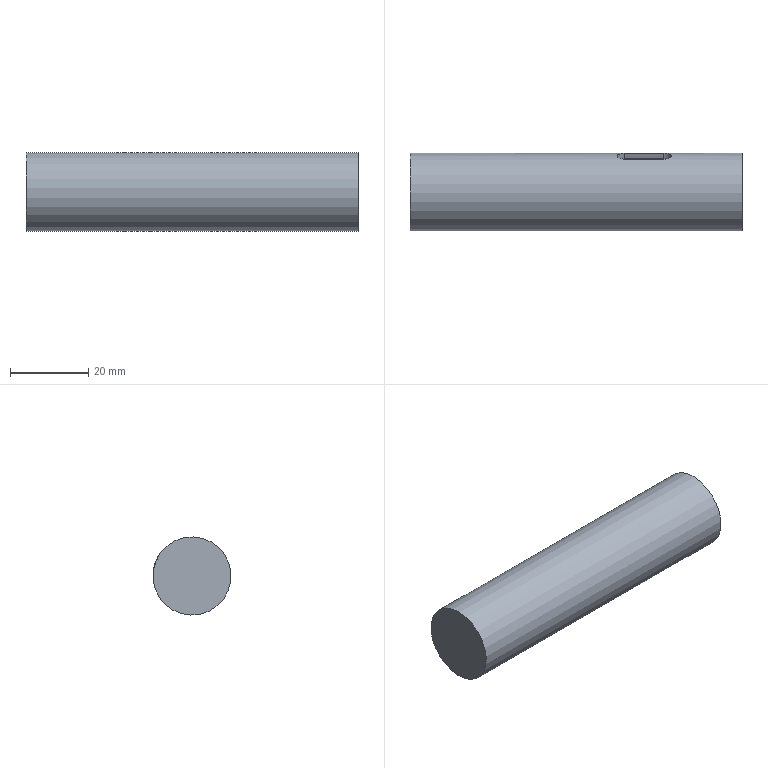Component | NX | CCJ-020 | 1 solid | 8 faces | box 85 x 20 x 20 mm | volume 26623 mm3 | plane 5 | cylinder 3 | commonest cylinder face diameters 4 x2 20 x1
STEP:
#1=CARTESIAN_POINT('',(0.,0.,0.));
#2=DIRECTION('',(0.,0.,1.));
#3=DIRECTION('',(1.,0.,0.));
#4=AXIS2_PLACEMENT_3D('',#1,#2,#3);
#5=CARTESIAN_POINT('',(26.329,34.242,-20.986));
#6=VERTEX_POINT('',#5);
#7=CARTESIAN_POINT('',(26.329,25.,-24.804));
#8=DIRECTION('',(-1.,0.,0.));
#9=DIRECTION('',(0.,0.9242,0.3818));
#10=AXIS2_PLACEMENT_3D('',#7,#8,#9);
#11=CIRCLE('',#10,10.);
#12=CARTESIAN_POINT('',(-58.671,25.,-24.804));
#13=DIRECTION('',(1.,0.,0.));
#14=DIRECTION('',(0.,-0.9242,-0.3818));
#15=AXIS2_PLACEMENT_3D('',#12,#13,#14);
#16=CYLINDRICAL_SURFACE('',#15,10.);
#17=CARTESIAN_POINT('',(9.425,85.));
#18=DIRECTION('',(-1.,0.));
#19=VECTOR('',#18,1.);
#20=LINE('',#17,#19);
#21=(GEOMETRIC_REPRESENTATION_CONTEXT(2)PARAMETRIC_REPRESENTATION_CONTEXT()REPRESENTATION_CONTEXT('',''));
#22=DEFINITIONAL_REPRESENTATION('',(#20),#21);
#23=PCURVE('',#16,#22);
#24=CARTESIAN_POINT('',(26.329,25.,-24.804));
#25=DIRECTION('',(-1.,0.,0.));
#26=DIRECTION('',(0.,0.9242,0.3818));
#27=AXIS2_PLACEMENT_3D('',#24,#25,#26);
#28=PLANE('',#27);
#29=CARTESIAN_POINT('',(0.,0.));
#30=DIRECTION('',(1.,0.));
#31=AXIS2_PLACEMENT_2D('',#29,#30);
#32=CIRCLE('',#31,10.);
#33=(GEOMETRIC_REPRESENTATION_CONTEXT(2)PARAMETRIC_REPRESENTATION_CONTEXT()REPRESENTATION_CONTEXT('',''));
#34=DEFINITIONAL_REPRESENTATION('',(#32),#33);
#35=PCURVE('',#28,#34);
#36=SURFACE_CURVE('',#11,(#23,#35),.PCURVE_S1.);
#37=EDGE_CURVE('',#6,#6,#36,.T.);
#38=ORIENTED_EDGE('',*,*,#37,.T.);
#39=CARTESIAN_POINT('',(8.329,34.242,-20.986));
#40=VERTEX_POINT('',#39);
#41=CARTESIAN_POINT('',(8.329,34.242,-20.986));
#42=CARTESIAN_POINT('',(26.329,34.242,-20.986));
#43=B_SPLINE_CURVE_WITH_KNOTS('',1,(#41,#42),.UNSPECIFIED.,.F.,.F.,(2,2),(67.,85.),.PIECEWISE_BEZIER_KNOTS.);
#44=CARTESIAN_POINT('',(3.142,0.));
#45=DIRECTION('',(0.,1.));
#46=VECTOR('',#45,1.);
#47=LINE('',#44,#46);
#48=(GEOMETRIC_REPRESENTATION_CONTEXT(2)PARAMETRIC_REPRESENTATION_CONTEXT()REPRESENTATION_CONTEXT('',''));
#49=DEFINITIONAL_REPRESENTATION('',(#47),#48);
#50=PCURVE('',#16,#49);
#51=CARTESIAN_POINT('',(9.425,0.));
#52=DIRECTION('',(0.,1.));
#53=VECTOR('',#52,1.);
#54=LINE('',#51,#53);
#55=(GEOMETRIC_REPRESENTATION_CONTEXT(2)PARAMETRIC_REPRESENTATION_CONTEXT()REPRESENTATION_CONTEXT('',''));
#56=DEFINITIONAL_REPRESENTATION('',(#54),#55);
#57=PCURVE('',#16,#56);
#58=SEAM_CURVE('',#43,(#50,#57),.PCURVE_S1.);
#59=EDGE_CURVE('',#40,#6,#58,.T.);
#60=ORIENTED_EDGE('',*,*,#59,.F.);
#61=CARTESIAN_POINT('',(6.329,33.292,-19.214));
#62=VERTEX_POINT('',#61);
#63=CARTESIAN_POINT('',(6.329,33.292,-19.214));
#64=CARTESIAN_POINT('',(6.55,33.292,-19.214));
#65=CARTESIAN_POINT('',(6.775,33.314,-19.246));
#66=CARTESIAN_POINT('',(6.983,33.354,-19.308));
#67=CARTESIAN_POINT('',(7.192,33.394,-19.369));
#68=CARTESIAN_POINT('',(7.391,33.455,-19.462));
#69=CARTESIAN_POINT('',(7.564,33.526,-19.579));
#70=CARTESIAN_POINT('',(7.739,33.599,-19.698));
#71=CARTESIAN_POINT('',(7.893,33.686,-19.846));
#72=CARTESIAN_POINT('',(8.014,33.777,-20.012));
#73=CARTESIAN_POINT('',(8.135,33.868,-20.179));
#74=CARTESIAN_POINT('',(8.225,33.966,-20.37));
#75=CARTESIAN_POINT('',(8.276,34.059,-20.569));
#76=CARTESIAN_POINT('',(8.327,34.151,-20.766));
#77=CARTESIAN_POINT('',(8.341,34.241,-20.976));
#78=CARTESIAN_POINT('',(8.318,34.321,-21.183));
#79=CARTESIAN_POINT('',(8.294,34.4,-21.387));
#80=CARTESIAN_POINT('',(8.234,34.472,-21.592));
#81=CARTESIAN_POINT('',(8.141,34.532,-21.782));
#82=CARTESIAN_POINT('',(8.047,34.593,-21.973));
#83=CARTESIAN_POINT('',(7.919,34.644,-22.154));
#84=CARTESIAN_POINT('',(7.766,34.684,-22.309));
#85=CARTESIAN_POINT('',(7.61,34.724,-22.466));
#86=CARTESIAN_POINT('',(7.424,34.755,-22.601));
#87=CARTESIAN_POINT('',(7.224,34.776,-22.7));
#88=CARTESIAN_POINT('',(7.023,34.798,-22.8));
#89=CARTESIAN_POINT('',(6.801,34.811,-22.868));
#90=CARTESIAN_POINT('',(6.577,34.816,-22.896));
#91=CARTESIAN_POINT('',(6.495,34.818,-22.906));
#92=CARTESIAN_POINT('',(6.412,34.819,-22.911));
#93=CARTESIAN_POINT('',(6.329,34.819,-22.911));
#94=B_SPLINE_CURVE_WITH_KNOTS('',3,(#63,#64,#65,#66,#67,#68,#69,#70,#71,#72,#73,#74,#75,#76,#77,#78,#79,#80,#81,#82,#83,#84,#85,#86,#87,#88,#89,#90,#91,#92,#93),.UNSPECIFIED.,.F.,.F.,(4,3,3,3,3,3,3,3,3,3,4),(0.,0.106,0.2118,0.319,0.4272,0.534,0.6392,0.745,0.8528,0.9608,1.),.UNSPECIFIED.);
#95=CARTESIAN_POINT('',(3.343,65.));
#96=CARTESIAN_POINT('',(3.343,65.047));
#97=CARTESIAN_POINT('',(3.343,65.143));
#98=CARTESIAN_POINT('',(3.341,65.285));
#99=CARTESIAN_POINT('',(3.338,65.427));
#100=CARTESIAN_POINT('',(3.335,65.565));
#101=CARTESIAN_POINT('',(3.33,65.7));
#102=CARTESIAN_POINT('',(3.325,65.832));
#103=CARTESIAN_POINT('',(3.318,65.96));
#104=CARTESIAN_POINT('',(3.311,66.083));
#105=CARTESIAN_POINT('',(3.302,66.2));
#106=CARTESIAN_POINT('',(3.293,66.31));
#107=CARTESIAN_POINT('',(3.284,66.415));
#108=CARTESIAN_POINT('',(3.273,66.512));
#109=CARTESIAN_POINT('',(3.262,66.602));
#110=CARTESIAN_POINT('',(3.25,66.683));
#111=CARTESIAN_POINT('',(3.238,66.756));
#112=CARTESIAN_POINT('',(3.225,66.82));
#113=CARTESIAN_POINT('',(3.212,66.875));
#114=CARTESIAN_POINT('',(3.198,66.92));
#115=CARTESIAN_POINT('',(3.184,66.956));
#116=CARTESIAN_POINT('',(3.17,66.981));
#117=CARTESIAN_POINT('',(3.156,66.996));
#118=CARTESIAN_POINT('',(3.142,67.002));
#119=CARTESIAN_POINT('',(3.127,66.997));
#120=CARTESIAN_POINT('',(3.113,66.981));
#121=CARTESIAN_POINT('',(3.099,66.956));
#122=CARTESIAN_POINT('',(3.085,66.92));
#123=CARTESIAN_POINT('',(3.072,66.875));
#124=CARTESIAN_POINT('',(3.058,66.821));
#125=CARTESIAN_POINT('',(3.046,66.757));
#126=CARTESIAN_POINT('',(3.033,66.684));
#127=CARTESIAN_POINT('',(3.021,66.603));
#128=CARTESIAN_POINT('',(3.01,66.513));
#129=CARTESIAN_POINT('',(3.,66.416));
#130=CARTESIAN_POINT('',(2.99,66.312));
#131=CARTESIAN_POINT('',(2.981,66.201));
#132=CARTESIAN_POINT('',(2.973,66.084));
#133=CARTESIAN_POINT('',(2.965,65.961));
#134=CARTESIAN_POINT('',(2.959,65.834));
#135=CARTESIAN_POINT('',(2.953,65.703));
#136=CARTESIAN_POINT('',(2.948,65.567));
#137=CARTESIAN_POINT('',(2.945,65.428));
#138=CARTESIAN_POINT('',(2.942,65.288));
#139=CARTESIAN_POINT('',(2.941,65.144));
#140=CARTESIAN_POINT('',(2.94,65.048));
#141=CARTESIAN_POINT('',(2.94,65.));
#142=B_SPLINE_CURVE_WITH_KNOTS('',3,(#95,#96,#97,#98,#99,#100,#101,#102,#103,#104,#105,#106,#107,#108,#109,#110,#111,#112,#113,#114,#115,#116,#117,#118,#119,#120,#121,#122,#123,#124,#125,#126,#127,#128,#129,#130,#131,#132,#133,#134,#135,#136,#137,#138,#139,#140,#141),.UNSPECIFIED.,.F.,.F.,(4,1,1,1,1,1,1,1,1,1,1,1,1,1,1,1,1,1,1,1,1,1,1,1,1,1,1,1,1,1,1,1,1,1,1,1,1,1,1,1,1,1,1,1,4),(0.,0.02273,0.04545,0.06818,0.09091,0.1136,0.1364,0.1591,0.1818,0.2045,0.2273,0.25,0.2727,0.2955,0.3182,0.3409,0.3636,0.3864,0.4091,0.4318,0.4545,0.4773,0.5,0.5227,0.5455,0.5682,0.5909,0.6136,0.6364,0.6591,0.6818,0.7045,0.7273,0.75,0.7727,0.7955,0.8182,0.8409,0.8636,0.8864,0.9091,0.9318,0.9545,0.9773,1.),.QUASI_UNIFORM_KNOTS.);
#143=(GEOMETRIC_REPRESENTATION_CONTEXT(2)PARAMETRIC_REPRESENTATION_CONTEXT()REPRESENTATION_CONTEXT('',''));
#144=DEFINITIONAL_REPRESENTATION('',(#142),#143);
#145=PCURVE('',#16,#144);
#146=CARTESIAN_POINT('',(6.329,38.863,-19.077));
#147=DIRECTION('',(0.,-0.9242,-0.3818));
#148=DIRECTION('',(-1.,0.,0.));
#149=AXIS2_PLACEMENT_3D('',#146,#147,#148);
#150=CYLINDRICAL_SURFACE('',#149,2.);
#151=CARTESIAN_POINT('',(4.712,5.202));
#152=CARTESIAN_POINT('',(3.142,5.));
#153=B_SPLINE_CURVE_WITH_KNOTS('',1,(#151,#152),.UNSPECIFIED.,.F.,.F.,(2,2),(0.,0.5001),.PIECEWISE_BEZIER_KNOTS.);
#154=(GEOMETRIC_REPRESENTATION_CONTEXT(2)PARAMETRIC_REPRESENTATION_CONTEXT()REPRESENTATION_CONTEXT('',''));
#155=DEFINITIONAL_REPRESENTATION('',(#153),#154);
#156=PCURVE('',#150,#155);
#157=SURFACE_CURVE('',#94,(#145,#156),.PCURVE_S1.);
#158=EDGE_CURVE('',#62,#40,#157,.T.);
#159=ORIENTED_EDGE('',*,*,#158,.F.);
#160=CARTESIAN_POINT('',(-3.671,33.292,-19.214));
#161=VERTEX_POINT('',#160);
#162=CARTESIAN_POINT('',(-58.671,33.292,-19.214));
#163=DIRECTION('',(1.,0.,0.));
#164=VECTOR('',#163,1.);
#165=LINE('',#162,#164);
#166=CARTESIAN_POINT('',(3.343,0.));
#167=DIRECTION('',(0.,1.));
#168=VECTOR('',#167,1.);
#169=LINE('',#166,#168);
#170=(GEOMETRIC_REPRESENTATION_CONTEXT(2)PARAMETRIC_REPRESENTATION_CONTEXT()REPRESENTATION_CONTEXT('',''));
#171=DEFINITIONAL_REPRESENTATION('',(#169),#170);
#172=PCURVE('',#16,#171);
#173=CARTESIAN_POINT('',(-3.671,38.1,-17.228));
#174=DIRECTION('',(0.,0.3818,-0.9242));
#175=DIRECTION('',(-1.,0.,0.));
#176=AXIS2_PLACEMENT_3D('',#173,#174,#175);
#177=PLANE('',#176);
#178=CARTESIAN_POINT('',(55.,-5.202));
#179=DIRECTION('',(-1.,0.));
#180=VECTOR('',#179,1.);
#181=LINE('',#178,#180);
#182=(GEOMETRIC_REPRESENTATION_CONTEXT(2)PARAMETRIC_REPRESENTATION_CONTEXT()REPRESENTATION_CONTEXT('',''));
#183=DEFINITIONAL_REPRESENTATION('',(#181),#182);
#184=PCURVE('',#177,#183);
#185=SURFACE_CURVE('',#165,(#172,#184),.PCURVE_S1.);
#186=EDGE_CURVE('',#161,#62,#185,.T.);
#187=ORIENTED_EDGE('',*,*,#186,.F.);
#188=CARTESIAN_POINT('',(-5.671,34.242,-20.986));
#189=VERTEX_POINT('',#188);
#190=CARTESIAN_POINT('',(-3.671,34.819,-22.911));
#191=CARTESIAN_POINT('',(-3.892,34.819,-22.911));
#192=CARTESIAN_POINT('',(-4.117,34.812,-22.873));
#193=CARTESIAN_POINT('',(-4.326,34.797,-22.801));
#194=CARTESIAN_POINT('',(-4.534,34.783,-22.729));
#195=CARTESIAN_POINT('',(-4.733,34.76,-22.621));
#196=CARTESIAN_POINT('',(-4.906,34.728,-22.487));
#197=CARTESIAN_POINT('',(-5.082,34.696,-22.352));
#198=CARTESIAN_POINT('',(-5.236,34.653,-22.186));
#199=CARTESIAN_POINT('',(-5.356,34.6,-22.004));
#200=CARTESIAN_POINT('',(-5.477,34.547,-21.821));
#201=CARTESIAN_POINT('',(-5.567,34.481,-21.617));
#202=CARTESIAN_POINT('',(-5.619,34.406,-21.41));
#203=CARTESIAN_POINT('',(-5.669,34.333,-21.206));
#204=CARTESIAN_POINT('',(-5.683,34.248,-20.993));
#205=CARTESIAN_POINT('',(-5.66,34.159,-20.79));
#206=CARTESIAN_POINT('',(-5.636,34.071,-20.59));
#207=CARTESIAN_POINT('',(-5.576,33.977,-20.394));
#208=CARTESIAN_POINT('',(-5.483,33.886,-20.217));
#209=CARTESIAN_POINT('',(-5.39,33.794,-20.039));
#210=CARTESIAN_POINT('',(-5.261,33.702,-19.875));
#211=CARTESIAN_POINT('',(-5.108,33.621,-19.737));
#212=CARTESIAN_POINT('',(-4.952,33.539,-19.597));
#213=CARTESIAN_POINT('',(-4.767,33.465,-19.48));
#214=CARTESIAN_POINT('',(-4.566,33.41,-19.394));
#215=CARTESIAN_POINT('',(-4.365,33.355,-19.308));
#216=CARTESIAN_POINT('',(-4.143,33.317,-19.251));
#217=CARTESIAN_POINT('',(-3.92,33.301,-19.228));
#218=CARTESIAN_POINT('',(-3.837,33.295,-19.219));
#219=CARTESIAN_POINT('',(-3.754,33.292,-19.214));
#220=CARTESIAN_POINT('',(-3.671,33.292,-19.214));
#221=B_SPLINE_CURVE_WITH_KNOTS('',3,(#190,#191,#192,#193,#194,#195,#196,#197,#198,#199,#200,#201,#202,#203,#204,#205,#206,#207,#208,#209,#210,#211,#212,#213,#214,#215,#216,#217,#218,#219,#220),.UNSPECIFIED.,.F.,.F.,(4,3,3,3,3,3,3,3,3,3,4),(0.,0.106,0.2118,0.319,0.4272,0.534,0.6392,0.745,0.8528,0.9608,1.),.UNSPECIFIED.);
#222=CARTESIAN_POINT('',(2.94,55.));
#223=CARTESIAN_POINT('',(2.94,54.953));
#224=CARTESIAN_POINT('',(2.941,54.857));
#225=CARTESIAN_POINT('',(2.942,54.715));
#226=CARTESIAN_POINT('',(2.945,54.573));
#227=CARTESIAN_POINT('',(2.948,54.435));
#228=CARTESIAN_POINT('',(2.953,54.3));
#229=CARTESIAN_POINT('',(2.959,54.168));
#230=CARTESIAN_POINT('',(2.965,54.04));
#231=CARTESIAN_POINT('',(2.972,53.917));
#232=CARTESIAN_POINT('',(2.981,53.8));
#233=CARTESIAN_POINT('',(2.99,53.69));
#234=CARTESIAN_POINT('',(3.,53.585));
#235=CARTESIAN_POINT('',(3.01,53.488));
#236=CARTESIAN_POINT('',(3.021,53.398));
#237=CARTESIAN_POINT('',(3.033,53.317));
#238=CARTESIAN_POINT('',(3.045,53.244));
#239=CARTESIAN_POINT('',(3.058,53.18));
#240=CARTESIAN_POINT('',(3.071,53.125));
#241=CARTESIAN_POINT('',(3.085,53.08));
#242=CARTESIAN_POINT('',(3.099,53.044));
#243=CARTESIAN_POINT('',(3.113,53.019));
#244=CARTESIAN_POINT('',(3.127,53.004));
#245=CARTESIAN_POINT('',(3.142,52.998));
#246=CARTESIAN_POINT('',(3.156,53.003));
#247=CARTESIAN_POINT('',(3.17,53.019));
#248=CARTESIAN_POINT('',(3.184,53.044));
#249=CARTESIAN_POINT('',(3.198,53.08));
#250=CARTESIAN_POINT('',(3.212,53.125));
#251=CARTESIAN_POINT('',(3.225,53.179));
#252=CARTESIAN_POINT('',(3.238,53.243));
#253=CARTESIAN_POINT('',(3.25,53.316));
#254=CARTESIAN_POINT('',(3.262,53.397));
#255=CARTESIAN_POINT('',(3.273,53.487));
#256=CARTESIAN_POINT('',(3.284,53.584));
#257=CARTESIAN_POINT('',(3.293,53.688));
#258=CARTESIAN_POINT('',(3.302,53.799));
#259=CARTESIAN_POINT('',(3.311,53.916));
#260=CARTESIAN_POINT('',(3.318,54.039));
#261=CARTESIAN_POINT('',(3.325,54.166));
#262=CARTESIAN_POINT('',(3.33,54.297));
#263=CARTESIAN_POINT('',(3.335,54.433));
#264=CARTESIAN_POINT('',(3.338,54.572));
#265=CARTESIAN_POINT('',(3.341,54.712));
#266=CARTESIAN_POINT('',(3.343,54.856));
#267=CARTESIAN_POINT('',(3.343,54.952));
#268=CARTESIAN_POINT('',(3.343,55.));
#269=B_SPLINE_CURVE_WITH_KNOTS('',3,(#222,#223,#224,#225,#226,#227,#228,#229,#230,#231,#232,#233,#234,#235,#236,#237,#238,#239,#240,#241,#242,#243,#244,#245,#246,#247,#248,#249,#250,#251,#252,#253,#254,#255,#256,#257,#258,#259,#260,#261,#262,#263,#264,#265,#266,#267,#268),.UNSPECIFIED.,.F.,.F.,(4,1,1,1,1,1,1,1,1,1,1,1,1,1,1,1,1,1,1,1,1,1,1,1,1,1,1,1,1,1,1,1,1,1,1,1,1,1,1,1,1,1,1,1,4),(0.,0.02273,0.04545,0.06818,0.09091,0.1136,0.1364,0.1591,0.1818,0.2045,0.2273,0.25,0.2727,0.2955,0.3182,0.3409,0.3636,0.3864,0.4091,0.4318,0.4545,0.4773,0.5,0.5227,0.5455,0.5682,0.5909,0.6136,0.6364,0.6591,0.6818,0.7045,0.7273,0.75,0.7727,0.7955,0.8182,0.8409,0.8636,0.8864,0.9091,0.9318,0.9545,0.9773,1.),.QUASI_UNIFORM_KNOTS.);
#270=(GEOMETRIC_REPRESENTATION_CONTEXT(2)PARAMETRIC_REPRESENTATION_CONTEXT()REPRESENTATION_CONTEXT('',''));
#271=DEFINITIONAL_REPRESENTATION('',(#269),#270);
#272=PCURVE('',#16,#271);
#273=CARTESIAN_POINT('',(-3.671,38.863,-19.077));
#274=DIRECTION('',(0.,-0.9242,-0.3818));
#275=DIRECTION('',(-1.,0.,0.));
#276=AXIS2_PLACEMENT_3D('',#273,#274,#275);
#277=CYLINDRICAL_SURFACE('',#276,2.);
#278=CARTESIAN_POINT('',(0.00000002,5.));
#279=CARTESIAN_POINT('',(-1.571,5.202));
#280=B_SPLINE_CURVE_WITH_KNOTS('',1,(#278,#279),.UNSPECIFIED.,.F.,.F.,(2,2),(0.5001,1.),.PIECEWISE_BEZIER_KNOTS.);
#281=(GEOMETRIC_REPRESENTATION_CONTEXT(2)PARAMETRIC_REPRESENTATION_CONTEXT()REPRESENTATION_CONTEXT('',''));
#282=DEFINITIONAL_REPRESENTATION('',(#280),#281);
#283=PCURVE('',#277,#282);
#284=SURFACE_CURVE('',#221,(#272,#283),.PCURVE_S1.);
#285=EDGE_CURVE('',#189,#161,#284,.T.);
#286=ORIENTED_EDGE('',*,*,#285,.F.);
#287=CARTESIAN_POINT('',(-58.671,34.242,-20.986));
#288=VERTEX_POINT('',#287);
#289=CARTESIAN_POINT('',(-58.671,34.242,-20.986));
#290=CARTESIAN_POINT('',(-5.671,34.242,-20.986));
#291=B_SPLINE_CURVE_WITH_KNOTS('',1,(#289,#290),.UNSPECIFIED.,.F.,.F.,(2,2),(0.,53.),.PIECEWISE_BEZIER_KNOTS.);
#292=CARTESIAN_POINT('',(3.142,0.));
#293=DIRECTION('',(0.,1.));
#294=VECTOR('',#293,1.);
#295=LINE('',#292,#294);
#296=(GEOMETRIC_REPRESENTATION_CONTEXT(2)PARAMETRIC_REPRESENTATION_CONTEXT()REPRESENTATION_CONTEXT('',''));
#297=DEFINITIONAL_REPRESENTATION('',(#295),#296);
#298=PCURVE('',#16,#297);
#299=CARTESIAN_POINT('',(9.425,0.));
#300=DIRECTION('',(0.,1.));
#301=VECTOR('',#300,1.);
#302=LINE('',#299,#301);
#303=(GEOMETRIC_REPRESENTATION_CONTEXT(2)PARAMETRIC_REPRESENTATION_CONTEXT()REPRESENTATION_CONTEXT('',''));
#304=DEFINITIONAL_REPRESENTATION('',(#302),#303);
#305=PCURVE('',#16,#304);
#306=SEAM_CURVE('',#291,(#298,#305),.PCURVE_S1.);
#307=EDGE_CURVE('',#288,#189,#306,.T.);
#308=ORIENTED_EDGE('',*,*,#307,.F.);
#309=CARTESIAN_POINT('',(-58.671,25.,-24.804));
#310=DIRECTION('',(-1.,0.,0.));
#311=DIRECTION('',(0.,0.9242,0.3818));
#312=AXIS2_PLACEMENT_3D('',#309,#310,#311);
#313=CIRCLE('',#312,10.);
#314=CARTESIAN_POINT('',(9.425,0.));
#315=DIRECTION('',(-1.,0.));
#316=VECTOR('',#315,1.);
#317=LINE('',#314,#316);
#318=(GEOMETRIC_REPRESENTATION_CONTEXT(2)PARAMETRIC_REPRESENTATION_CONTEXT()REPRESENTATION_CONTEXT('',''));
#319=DEFINITIONAL_REPRESENTATION('',(#317),#318);
#320=PCURVE('',#16,#319);
#321=CARTESIAN_POINT('',(-58.671,25.,-24.804));
#322=DIRECTION('',(-1.,0.,0.));
#323=DIRECTION('',(0.,0.9242,0.3818));
#324=AXIS2_PLACEMENT_3D('',#321,#322,#323);
#325=PLANE('',#324);
#326=CARTESIAN_POINT('',(0.,0.));
#327=DIRECTION('',(1.,0.));
#328=AXIS2_PLACEMENT_2D('',#326,#327);
#329=CIRCLE('',#328,10.);
#330=(GEOMETRIC_REPRESENTATION_CONTEXT(2)PARAMETRIC_REPRESENTATION_CONTEXT()REPRESENTATION_CONTEXT('',''));
#331=DEFINITIONAL_REPRESENTATION('',(#329),#330);
#332=PCURVE('',#325,#331);
#333=SURFACE_CURVE('',#313,(#320,#332),.PCURVE_S1.);
#334=EDGE_CURVE('',#288,#288,#333,.T.);
#335=ORIENTED_EDGE('',*,*,#334,.F.);
#336=ORIENTED_EDGE('',*,*,#307,.T.);
#337=CARTESIAN_POINT('',(-3.671,34.819,-22.911));
#338=VERTEX_POINT('',#337);
#339=CARTESIAN_POINT('',(-3.671,34.819,-22.911));
#340=CARTESIAN_POINT('',(-3.892,34.819,-22.911));
#341=CARTESIAN_POINT('',(-4.117,34.812,-22.873));
#342=CARTESIAN_POINT('',(-4.326,34.797,-22.801));
#343=CARTESIAN_POINT('',(-4.534,34.783,-22.729));
#344=CARTESIAN_POINT('',(-4.733,34.76,-22.621));
#345=CARTESIAN_POINT('',(-4.906,34.728,-22.487));
#346=CARTESIAN_POINT('',(-5.082,34.696,-22.352));
#347=CARTESIAN_POINT('',(-5.236,34.653,-22.186));
#348=CARTESIAN_POINT('',(-5.356,34.6,-22.004));
#349=CARTESIAN_POINT('',(-5.477,34.547,-21.821));
#350=CARTESIAN_POINT('',(-5.567,34.481,-21.617));
#351=CARTESIAN_POINT('',(-5.619,34.406,-21.41));
#352=CARTESIAN_POINT('',(-5.669,34.333,-21.206));
#353=CARTESIAN_POINT('',(-5.683,34.248,-20.993));
#354=CARTESIAN_POINT('',(-5.66,34.159,-20.79));
#355=CARTESIAN_POINT('',(-5.636,34.071,-20.59));
#356=CARTESIAN_POINT('',(-5.576,33.977,-20.394));
#357=CARTESIAN_POINT('',(-5.483,33.886,-20.217));
#358=CARTESIAN_POINT('',(-5.39,33.794,-20.039));
#359=CARTESIAN_POINT('',(-5.261,33.702,-19.875));
#360=CARTESIAN_POINT('',(-5.108,33.621,-19.737));
#361=CARTESIAN_POINT('',(-4.952,33.539,-19.597));
#362=CARTESIAN_POINT('',(-4.767,33.465,-19.48));
#363=CARTESIAN_POINT('',(-4.566,33.41,-19.394));
#364=CARTESIAN_POINT('',(-4.365,33.355,-19.308));
#365=CARTESIAN_POINT('',(-4.143,33.317,-19.251));
#366=CARTESIAN_POINT('',(-3.92,33.301,-19.228));
#367=CARTESIAN_POINT('',(-3.837,33.295,-19.219));
#368=CARTESIAN_POINT('',(-3.754,33.292,-19.214));
#369=CARTESIAN_POINT('',(-3.671,33.292,-19.214));
#370=B_SPLINE_CURVE_WITH_KNOTS('',3,(#339,#340,#341,#342,#343,#344,#345,#346,#347,#348,#349,#350,#351,#352,#353,#354,#355,#356,#357,#358,#359,#360,#361,#362,#363,#364,#365,#366,#367,#368,#369),.UNSPECIFIED.,.F.,.F.,(4,3,3,3,3,3,3,3,3,3,4),(0.,0.106,0.2118,0.319,0.4272,0.534,0.6392,0.745,0.8528,0.9608,1.),.UNSPECIFIED.);
#371=CARTESIAN_POINT('',(9.223,55.));
#372=CARTESIAN_POINT('',(9.223,54.953));
#373=CARTESIAN_POINT('',(9.224,54.857));
#374=CARTESIAN_POINT('',(9.225,54.715));
#375=CARTESIAN_POINT('',(9.228,54.573));
#376=CARTESIAN_POINT('',(9.232,54.435));
#377=CARTESIAN_POINT('',(9.236,54.3));
#378=CARTESIAN_POINT('',(9.242,54.168));
#379=CARTESIAN_POINT('',(9.248,54.04));
#380=CARTESIAN_POINT('',(9.256,53.917));
#381=CARTESIAN_POINT('',(9.264,53.8));
#382=CARTESIAN_POINT('',(9.273,53.69));
#383=CARTESIAN_POINT('',(9.283,53.585));
#384=CARTESIAN_POINT('',(9.293,53.488));
#385=CARTESIAN_POINT('',(9.304,53.398));
#386=CARTESIAN_POINT('',(9.316,53.317));
#387=CARTESIAN_POINT('',(9.329,53.244));
#388=CARTESIAN_POINT('',(9.341,53.18));
#389=CARTESIAN_POINT('',(9.355,53.125));
#390=CARTESIAN_POINT('',(9.368,53.08));
#391=CARTESIAN_POINT('',(9.382,53.044));
#392=CARTESIAN_POINT('',(9.396,53.019));
#393=CARTESIAN_POINT('',(9.41,53.004));
#394=CARTESIAN_POINT('',(9.425,52.998));
#395=CARTESIAN_POINT('',(9.439,53.003));
#396=CARTESIAN_POINT('',(9.453,53.019));
#397=CARTESIAN_POINT('',(9.467,53.044));
#398=CARTESIAN_POINT('',(9.481,53.08));
#399=CARTESIAN_POINT('',(9.495,53.125));
#400=CARTESIAN_POINT('',(9.508,53.179));
#401=CARTESIAN_POINT('',(9.521,53.243));
#402=CARTESIAN_POINT('',(9.533,53.316));
#403=CARTESIAN_POINT('',(9.545,53.397));
#404=CARTESIAN_POINT('',(9.556,53.487));
#405=CARTESIAN_POINT('',(9.567,53.584));
#406=CARTESIAN_POINT('',(9.576,53.688));
#407=CARTESIAN_POINT('',(9.586,53.799));
#408=CARTESIAN_POINT('',(9.594,53.916));
#409=CARTESIAN_POINT('',(9.601,54.039));
#410=CARTESIAN_POINT('',(9.608,54.166));
#411=CARTESIAN_POINT('',(9.613,54.297));
#412=CARTESIAN_POINT('',(9.618,54.433));
#413=CARTESIAN_POINT('',(9.622,54.572));
#414=CARTESIAN_POINT('',(9.624,54.712));
#415=CARTESIAN_POINT('',(9.626,54.856));
#416=CARTESIAN_POINT('',(9.626,54.952));
#417=CARTESIAN_POINT('',(9.626,55.));
#418=B_SPLINE_CURVE_WITH_KNOTS('',3,(#371,#372,#373,#374,#375,#376,#377,#378,#379,#380,#381,#382,#383,#384,#385,#386,#387,#388,#389,#390,#391,#392,#393,#394,#395,#396,#397,#398,#399,#400,#401,#402,#403,#404,#405,#406,#407,#408,#409,#410,#411,#412,#413,#414,#415,#416,#417),.UNSPECIFIED.,.F.,.F.,(4,1,1,1,1,1,1,1,1,1,1,1,1,1,1,1,1,1,1,1,1,1,1,1,1,1,1,1,1,1,1,1,1,1,1,1,1,1,1,1,1,1,1,1,4),(0.,0.02273,0.04545,0.06818,0.09091,0.1136,0.1364,0.1591,0.1818,0.2045,0.2273,0.25,0.2727,0.2955,0.3182,0.3409,0.3636,0.3864,0.4091,0.4318,0.4545,0.4773,0.5,0.5227,0.5455,0.5682,0.5909,0.6136,0.6364,0.6591,0.6818,0.7045,0.7273,0.75,0.7727,0.7955,0.8182,0.8409,0.8636,0.8864,0.9091,0.9318,0.9545,0.9773,1.),.QUASI_UNIFORM_KNOTS.);
#419=(GEOMETRIC_REPRESENTATION_CONTEXT(2)PARAMETRIC_REPRESENTATION_CONTEXT()REPRESENTATION_CONTEXT('',''));
#420=DEFINITIONAL_REPRESENTATION('',(#418),#419);
#421=PCURVE('',#16,#420);
#422=CARTESIAN_POINT('',(1.571,5.202));
#423=CARTESIAN_POINT('',(0.00000002,5.));
#424=B_SPLINE_CURVE_WITH_KNOTS('',1,(#422,#423),.UNSPECIFIED.,.F.,.F.,(2,2),(0.,0.5001),.PIECEWISE_BEZIER_KNOTS.);
#425=(GEOMETRIC_REPRESENTATION_CONTEXT(2)PARAMETRIC_REPRESENTATION_CONTEXT()REPRESENTATION_CONTEXT('',''));
#426=DEFINITIONAL_REPRESENTATION('',(#424),#425);
#427=PCURVE('',#277,#426);
#428=SURFACE_CURVE('',#370,(#421,#427),.PCURVE_S1.);
#429=EDGE_CURVE('',#338,#189,#428,.T.);
#430=ORIENTED_EDGE('',*,*,#429,.F.);
#431=CARTESIAN_POINT('',(6.329,34.819,-22.911));
#432=VERTEX_POINT('',#431);
#433=CARTESIAN_POINT('',(-58.671,34.819,-22.911));
#434=DIRECTION('',(-1.,0.,0.));
#435=VECTOR('',#434,1.);
#436=LINE('',#433,#435);
#437=CARTESIAN_POINT('',(9.223,0.));
#438=DIRECTION('',(0.,-1.));
#439=VECTOR('',#438,1.);
#440=LINE('',#437,#439);
#441=(GEOMETRIC_REPRESENTATION_CONTEXT(2)PARAMETRIC_REPRESENTATION_CONTEXT()REPRESENTATION_CONTEXT('',''));
#442=DEFINITIONAL_REPRESENTATION('',(#440),#441);
#443=PCURVE('',#16,#442);
#444=CARTESIAN_POINT('',(6.329,39.627,-20.925));
#445=DIRECTION('',(0.,-0.3818,0.9242));
#446=DIRECTION('',(1.,0.,0.));
#447=AXIS2_PLACEMENT_3D('',#444,#445,#446);
#448=PLANE('',#447);
#449=CARTESIAN_POINT('',(-65.,-5.202));
#450=DIRECTION('',(-1.,0.));
#451=VECTOR('',#450,1.);
#452=LINE('',#449,#451);
#453=(GEOMETRIC_REPRESENTATION_CONTEXT(2)PARAMETRIC_REPRESENTATION_CONTEXT()REPRESENTATION_CONTEXT('',''));
#454=DEFINITIONAL_REPRESENTATION('',(#452),#453);
#455=PCURVE('',#448,#454);
#456=SURFACE_CURVE('',#436,(#443,#455),.PCURVE_S1.);
#457=EDGE_CURVE('',#432,#338,#456,.T.);
#458=ORIENTED_EDGE('',*,*,#457,.F.);
#459=CARTESIAN_POINT('',(6.329,33.292,-19.214));
#460=CARTESIAN_POINT('',(6.55,33.292,-19.214));
#461=CARTESIAN_POINT('',(6.775,33.314,-19.246));
#462=CARTESIAN_POINT('',(6.983,33.354,-19.308));
#463=CARTESIAN_POINT('',(7.192,33.394,-19.369));
#464=CARTESIAN_POINT('',(7.391,33.455,-19.462));
#465=CARTESIAN_POINT('',(7.564,33.526,-19.579));
#466=CARTESIAN_POINT('',(7.739,33.599,-19.698));
#467=CARTESIAN_POINT('',(7.893,33.686,-19.846));
#468=CARTESIAN_POINT('',(8.014,33.777,-20.012));
#469=CARTESIAN_POINT('',(8.135,33.868,-20.179));
#470=CARTESIAN_POINT('',(8.225,33.966,-20.37));
#471=CARTESIAN_POINT('',(8.276,34.059,-20.569));
#472=CARTESIAN_POINT('',(8.327,34.151,-20.766));
#473=CARTESIAN_POINT('',(8.341,34.241,-20.976));
#474=CARTESIAN_POINT('',(8.318,34.321,-21.183));
#475=CARTESIAN_POINT('',(8.294,34.4,-21.387));
#476=CARTESIAN_POINT('',(8.234,34.472,-21.592));
#477=CARTESIAN_POINT('',(8.141,34.532,-21.782));
#478=CARTESIAN_POINT('',(8.047,34.593,-21.973));
#479=CARTESIAN_POINT('',(7.919,34.644,-22.154));
#480=CARTESIAN_POINT('',(7.766,34.684,-22.309));
#481=CARTESIAN_POINT('',(7.61,34.724,-22.466));
#482=CARTESIAN_POINT('',(7.424,34.755,-22.601));
#483=CARTESIAN_POINT('',(7.224,34.776,-22.7));
#484=CARTESIAN_POINT('',(7.023,34.798,-22.8));
#485=CARTESIAN_POINT('',(6.801,34.811,-22.868));
#486=CARTESIAN_POINT('',(6.577,34.816,-22.896));
#487=CARTESIAN_POINT('',(6.495,34.818,-22.906));
#488=CARTESIAN_POINT('',(6.412,34.819,-22.911));
#489=CARTESIAN_POINT('',(6.329,34.819,-22.911));
#490=B_SPLINE_CURVE_WITH_KNOTS('',3,(#459,#460,#461,#462,#463,#464,#465,#466,#467,#468,#469,#470,#471,#472,#473,#474,#475,#476,#477,#478,#479,#480,#481,#482,#483,#484,#485,#486,#487,#488,#489),.UNSPECIFIED.,.F.,.F.,(4,3,3,3,3,3,3,3,3,3,4),(0.,0.106,0.2118,0.319,0.4272,0.534,0.6392,0.745,0.8528,0.9608,1.),.UNSPECIFIED.);
#491=CARTESIAN_POINT('',(9.626,65.));
#492=CARTESIAN_POINT('',(9.626,65.047));
#493=CARTESIAN_POINT('',(9.626,65.143));
#494=CARTESIAN_POINT('',(9.624,65.285));
#495=CARTESIAN_POINT('',(9.622,65.427));
#496=CARTESIAN_POINT('',(9.618,65.565));
#497=CARTESIAN_POINT('',(9.613,65.7));
#498=CARTESIAN_POINT('',(9.608,65.832));
#499=CARTESIAN_POINT('',(9.601,65.96));
#500=CARTESIAN_POINT('',(9.594,66.083));
#501=CARTESIAN_POINT('',(9.586,66.2));
#502=CARTESIAN_POINT('',(9.577,66.31));
#503=CARTESIAN_POINT('',(9.567,66.415));
#504=CARTESIAN_POINT('',(9.556,66.512));
#505=CARTESIAN_POINT('',(9.545,66.602));
#506=CARTESIAN_POINT('',(9.533,66.683));
#507=CARTESIAN_POINT('',(9.521,66.756));
#508=CARTESIAN_POINT('',(9.508,66.82));
#509=CARTESIAN_POINT('',(9.495,66.875));
#510=CARTESIAN_POINT('',(9.481,66.92));
#511=CARTESIAN_POINT('',(9.468,66.956));
#512=CARTESIAN_POINT('',(9.453,66.981));
#513=CARTESIAN_POINT('',(9.439,66.996));
#514=CARTESIAN_POINT('',(9.425,67.002));
#515=CARTESIAN_POINT('',(9.411,66.997));
#516=CARTESIAN_POINT('',(9.396,66.981));
#517=CARTESIAN_POINT('',(9.382,66.956));
#518=CARTESIAN_POINT('',(9.368,66.92));
#519=CARTESIAN_POINT('',(9.355,66.875));
#520=CARTESIAN_POINT('',(9.342,66.821));
#521=CARTESIAN_POINT('',(9.329,66.757));
#522=CARTESIAN_POINT('',(9.316,66.684));
#523=CARTESIAN_POINT('',(9.305,66.603));
#524=CARTESIAN_POINT('',(9.293,66.513));
#525=CARTESIAN_POINT('',(9.283,66.416));
#526=CARTESIAN_POINT('',(9.273,66.312));
#527=CARTESIAN_POINT('',(9.264,66.201));
#528=CARTESIAN_POINT('',(9.256,66.084));
#529=CARTESIAN_POINT('',(9.248,65.961));
#530=CARTESIAN_POINT('',(9.242,65.834));
#531=CARTESIAN_POINT('',(9.236,65.703));
#532=CARTESIAN_POINT('',(9.232,65.567));
#533=CARTESIAN_POINT('',(9.228,65.428));
#534=CARTESIAN_POINT('',(9.225,65.288));
#535=CARTESIAN_POINT('',(9.224,65.144));
#536=CARTESIAN_POINT('',(9.223,65.048));
#537=CARTESIAN_POINT('',(9.223,65.));
#538=B_SPLINE_CURVE_WITH_KNOTS('',3,(#491,#492,#493,#494,#495,#496,#497,#498,#499,#500,#501,#502,#503,#504,#505,#506,#507,#508,#509,#510,#511,#512,#513,#514,#515,#516,#517,#518,#519,#520,#521,#522,#523,#524,#525,#526,#527,#528,#529,#530,#531,#532,#533,#534,#535,#536,#537),.UNSPECIFIED.,.F.,.F.,(4,1,1,1,1,1,1,1,1,1,1,1,1,1,1,1,1,1,1,1,1,1,1,1,1,1,1,1,1,1,1,1,1,1,1,1,1,1,1,1,1,1,1,1,4),(0.,0.02273,0.04545,0.06818,0.09091,0.1136,0.1364,0.1591,0.1818,0.2045,0.2273,0.25,0.2727,0.2955,0.3182,0.3409,0.3636,0.3864,0.4091,0.4318,0.4545,0.4773,0.5,0.5227,0.5455,0.5682,0.5909,0.6136,0.6364,0.6591,0.6818,0.7045,0.7273,0.75,0.7727,0.7955,0.8182,0.8409,0.8636,0.8864,0.9091,0.9318,0.9545,0.9773,1.),.QUASI_UNIFORM_KNOTS.);
#539=(GEOMETRIC_REPRESENTATION_CONTEXT(2)PARAMETRIC_REPRESENTATION_CONTEXT()REPRESENTATION_CONTEXT('',''));
#540=DEFINITIONAL_REPRESENTATION('',(#538),#539);
#541=PCURVE('',#16,#540);
#542=CARTESIAN_POINT('',(3.142,5.));
#543=CARTESIAN_POINT('',(1.571,5.202));
#544=B_SPLINE_CURVE_WITH_KNOTS('',1,(#542,#543),.UNSPECIFIED.,.F.,.F.,(2,2),(0.5001,1.),.PIECEWISE_BEZIER_KNOTS.);
#545=(GEOMETRIC_REPRESENTATION_CONTEXT(2)PARAMETRIC_REPRESENTATION_CONTEXT()REPRESENTATION_CONTEXT('',''));
#546=DEFINITIONAL_REPRESENTATION('',(#544),#545);
#547=PCURVE('',#150,#546);
#548=SURFACE_CURVE('',#490,(#541,#547),.PCURVE_S1.);
#549=EDGE_CURVE('',#40,#432,#548,.T.);
#550=ORIENTED_EDGE('',*,*,#549,.F.);
#551=ORIENTED_EDGE('',*,*,#59,.T.);
#552=EDGE_LOOP('',(#38,#60,#159,#187,#286,#308,#335,#336,#430,#458,#550,#551));
#553=FACE_BOUND('',#552,.T.);
#554=ADVANCED_FACE('',(#553),#16,.T.);
#555=ORIENTED_EDGE('',*,*,#334,.T.);
#556=EDGE_LOOP('',(#555));
#557=FACE_BOUND('',#556,.T.);
#558=ADVANCED_FACE('',(#557),#325,.T.);
#559=ORIENTED_EDGE('',*,*,#37,.F.);
#560=EDGE_LOOP('',(#559));
#561=FACE_BOUND('',#560,.T.);
#562=ADVANCED_FACE('',(#561),#28,.F.);
#563=ORIENTED_EDGE('',*,*,#186,.T.);
#564=CARTESIAN_POINT('',(6.329,32.,-19.748));
#565=VERTEX_POINT('',#564);
#566=CARTESIAN_POINT('',(6.329,38.1,-17.228));
#567=DIRECTION('',(0.,0.9242,0.3818));
#568=VECTOR('',#567,1.);
#569=LINE('',#566,#568);
#570=CARTESIAN_POINT('',(-10.,0.));
#571=DIRECTION('',(0.,1.));
#572=VECTOR('',#571,1.);
#573=LINE('',#570,#572);
#574=(GEOMETRIC_REPRESENTATION_CONTEXT(2)PARAMETRIC_REPRESENTATION_CONTEXT()REPRESENTATION_CONTEXT('',''));
#575=DEFINITIONAL_REPRESENTATION('',(#573),#574);
#576=PCURVE('',#177,#575);
#577=CARTESIAN_POINT('',(4.712,0.));
#578=DIRECTION('',(0.,-1.));
#579=VECTOR('',#578,1.);
#580=LINE('',#577,#579);
#581=(GEOMETRIC_REPRESENTATION_CONTEXT(2)PARAMETRIC_REPRESENTATION_CONTEXT()REPRESENTATION_CONTEXT('',''));
#582=DEFINITIONAL_REPRESENTATION('',(#580),#581);
#583=PCURVE('',#150,#582);
#584=SURFACE_CURVE('',#569,(#576,#583),.PCURVE_S1.);
#585=EDGE_CURVE('',#565,#62,#584,.T.);
#586=ORIENTED_EDGE('',*,*,#585,.F.);
#587=CARTESIAN_POINT('',(-3.671,32.,-19.748));
#588=VERTEX_POINT('',#587);
#589=CARTESIAN_POINT('',(-3.671,32.,-19.748));
#590=DIRECTION('',(-1.,0.,0.));
#591=VECTOR('',#590,1.);
#592=LINE('',#589,#591);
#593=CARTESIAN_POINT('',(0.,-6.6));
#594=DIRECTION('',(1.,0.));
#595=VECTOR('',#594,1.);
#596=LINE('',#593,#595);
#597=(GEOMETRIC_REPRESENTATION_CONTEXT(2)PARAMETRIC_REPRESENTATION_CONTEXT()REPRESENTATION_CONTEXT('',''));
#598=DEFINITIONAL_REPRESENTATION('',(#596),#597);
#599=PCURVE('',#177,#598);
#600=CARTESIAN_POINT('',(6.329,32.763,-21.597));
#601=DIRECTION('',(0.,0.9242,0.3818));
#602=DIRECTION('',(1.,0.,0.));
#603=AXIS2_PLACEMENT_3D('',#600,#601,#602);
#604=PLANE('',#603);
#605=CARTESIAN_POINT('',(-10.,-2.));
#606=DIRECTION('',(-1.,0.));
#607=VECTOR('',#606,1.);
#608=LINE('',#605,#607);
#609=(GEOMETRIC_REPRESENTATION_CONTEXT(2)PARAMETRIC_REPRESENTATION_CONTEXT()REPRESENTATION_CONTEXT('',''));
#610=DEFINITIONAL_REPRESENTATION('',(#608),#609);
#611=PCURVE('',#604,#610);
#612=SURFACE_CURVE('',#592,(#599,#611),.PCURVE_S1.);
#613=EDGE_CURVE('',#565,#588,#612,.T.);
#614=ORIENTED_EDGE('',*,*,#613,.T.);
#615=CARTESIAN_POINT('',(-3.671,38.1,-17.228));
#616=DIRECTION('',(0.,0.9242,0.3818));
#617=VECTOR('',#616,1.);
#618=LINE('',#615,#617);
#619=CARTESIAN_POINT('',(0.,0.));
#620=DIRECTION('',(0.,1.));
#621=VECTOR('',#620,1.);
#622=LINE('',#619,#621);
#623=(GEOMETRIC_REPRESENTATION_CONTEXT(2)PARAMETRIC_REPRESENTATION_CONTEXT()REPRESENTATION_CONTEXT('',''));
#624=DEFINITIONAL_REPRESENTATION('',(#622),#623);
#625=PCURVE('',#177,#624);
#626=CARTESIAN_POINT('',(-1.571,0.));
#627=DIRECTION('',(0.,-1.));
#628=VECTOR('',#627,1.);
#629=LINE('',#626,#628);
#630=(GEOMETRIC_REPRESENTATION_CONTEXT(2)PARAMETRIC_REPRESENTATION_CONTEXT()REPRESENTATION_CONTEXT('',''));
#631=DEFINITIONAL_REPRESENTATION('',(#629),#630);
#632=PCURVE('',#277,#631);
#633=SURFACE_CURVE('',#618,(#625,#632),.PCURVE_S1.);
#634=EDGE_CURVE('',#588,#161,#633,.T.);
#635=ORIENTED_EDGE('',*,*,#634,.T.);
#636=EDGE_LOOP('',(#563,#586,#614,#635));
#637=FACE_BOUND('',#636,.T.);
#638=ADVANCED_FACE('',(#637),#177,.T.);
#639=ORIENTED_EDGE('',*,*,#585,.F.);
#640=CARTESIAN_POINT('',(6.329,33.527,-23.445));
#641=VERTEX_POINT('',#640);
#642=CARTESIAN_POINT('',(6.329,32.763,-21.597));
#643=DIRECTION('',(0.,-0.9242,-0.3818));
#644=DIRECTION('',(0.,0.3818,-0.9242));
#645=AXIS2_PLACEMENT_3D('',#642,#643,#644);
#646=CIRCLE('',#645,2.);
#647=CARTESIAN_POINT('',(1.571,6.6));
#648=DIRECTION('',(1.,0.));
#649=VECTOR('',#648,1.);
#650=LINE('',#647,#649);
#651=(GEOMETRIC_REPRESENTATION_CONTEXT(2)PARAMETRIC_REPRESENTATION_CONTEXT()REPRESENTATION_CONTEXT('',''));
#652=DEFINITIONAL_REPRESENTATION('',(#650),#651);
#653=PCURVE('',#150,#652);
#654=CARTESIAN_POINT('',(0.,2.));
#655=CARTESIAN_POINT('',(3.464,2.));
#656=CARTESIAN_POINT('',(1.732,-1.));
#657=CARTESIAN_POINT('',(0.,-4.));
#658=CARTESIAN_POINT('',(-1.732,-1.));
#659=CARTESIAN_POINT('',(-3.464,2.));
#660=CARTESIAN_POINT('',(0.,2.));
#661=(BOUNDED_CURVE()B_SPLINE_CURVE(2,(#654,#655,#656,#657,#658,#659,#660),.UNSPECIFIED.,.T.,.F.)B_SPLINE_CURVE_WITH_KNOTS((1,2,2,2,2,1),(-2.094,0.,2.094,4.189,6.283,8.378),.UNSPECIFIED.)CURVE()GEOMETRIC_REPRESENTATION_ITEM()RATIONAL_B_SPLINE_CURVE((1.,0.5,1.,0.5,1.,0.5,1.))REPRESENTATION_ITEM(''));
#662=(GEOMETRIC_REPRESENTATION_CONTEXT(2)PARAMETRIC_REPRESENTATION_CONTEXT()REPRESENTATION_CONTEXT('',''));
#663=DEFINITIONAL_REPRESENTATION('',(#661),#662);
#664=PCURVE('',#604,#663);
#665=SURFACE_CURVE('',#646,(#653,#664),.PCURVE_S1.);
#666=EDGE_CURVE('',#641,#565,#665,.T.);
#667=ORIENTED_EDGE('',*,*,#666,.F.);
#668=CARTESIAN_POINT('',(6.329,39.627,-20.925));
#669=DIRECTION('',(0.,0.9242,0.3818));
#670=VECTOR('',#669,1.);
#671=LINE('',#668,#670);
#672=CARTESIAN_POINT('',(1.571,0.));
#673=DIRECTION('',(0.,-1.));
#674=VECTOR('',#673,1.);
#675=LINE('',#672,#674);
#676=(GEOMETRIC_REPRESENTATION_CONTEXT(2)PARAMETRIC_REPRESENTATION_CONTEXT()REPRESENTATION_CONTEXT('',''));
#677=DEFINITIONAL_REPRESENTATION('',(#675),#676);
#678=PCURVE('',#150,#677);
#679=CARTESIAN_POINT('',(0.,0.));
#680=DIRECTION('',(0.,1.));
#681=VECTOR('',#680,1.);
#682=LINE('',#679,#681);
#683=(GEOMETRIC_REPRESENTATION_CONTEXT(2)PARAMETRIC_REPRESENTATION_CONTEXT()REPRESENTATION_CONTEXT('',''));
#684=DEFINITIONAL_REPRESENTATION('',(#682),#683);
#685=PCURVE('',#448,#684);
#686=SURFACE_CURVE('',#671,(#678,#685),.PCURVE_S1.);
#687=EDGE_CURVE('',#641,#432,#686,.T.);
#688=ORIENTED_EDGE('',*,*,#687,.T.);
#689=ORIENTED_EDGE('',*,*,#549,.F.);
#690=ORIENTED_EDGE('',*,*,#158,.F.);
#691=EDGE_LOOP('',(#639,#667,#688,#689,#690));
#692=FACE_BOUND('',#691,.F.);
#693=ADVANCED_FACE('',(#692),#150,.F.);
#694=ORIENTED_EDGE('',*,*,#457,.T.);
#695=CARTESIAN_POINT('',(-3.671,33.527,-23.445));
#696=VERTEX_POINT('',#695);
#697=CARTESIAN_POINT('',(-3.671,39.627,-20.925));
#698=DIRECTION('',(0.,0.9242,0.3818));
#699=VECTOR('',#698,1.);
#700=LINE('',#697,#699);
#701=CARTESIAN_POINT('',(-10.,0.));
#702=DIRECTION('',(0.,1.));
#703=VECTOR('',#702,1.);
#704=LINE('',#701,#703);
#705=(GEOMETRIC_REPRESENTATION_CONTEXT(2)PARAMETRIC_REPRESENTATION_CONTEXT()REPRESENTATION_CONTEXT('',''));
#706=DEFINITIONAL_REPRESENTATION('',(#704),#705);
#707=PCURVE('',#448,#706);
#708=CARTESIAN_POINT('',(1.571,0.));
#709=DIRECTION('',(0.,-1.));
#710=VECTOR('',#709,1.);
#711=LINE('',#708,#710);
#712=(GEOMETRIC_REPRESENTATION_CONTEXT(2)PARAMETRIC_REPRESENTATION_CONTEXT()REPRESENTATION_CONTEXT('',''));
#713=DEFINITIONAL_REPRESENTATION('',(#711),#712);
#714=PCURVE('',#277,#713);
#715=SURFACE_CURVE('',#700,(#707,#714),.PCURVE_S1.);
#716=EDGE_CURVE('',#696,#338,#715,.T.);
#717=ORIENTED_EDGE('',*,*,#716,.F.);
#718=CARTESIAN_POINT('',(6.329,33.527,-23.445));
#719=DIRECTION('',(1.,0.,0.));
#720=VECTOR('',#719,1.);
#721=LINE('',#718,#720);
#722=CARTESIAN_POINT('',(0.,-6.6));
#723=DIRECTION('',(1.,0.));
#724=VECTOR('',#723,1.);
#725=LINE('',#722,#724);
#726=(GEOMETRIC_REPRESENTATION_CONTEXT(2)PARAMETRIC_REPRESENTATION_CONTEXT()REPRESENTATION_CONTEXT('',''));
#727=DEFINITIONAL_REPRESENTATION('',(#725),#726);
#728=PCURVE('',#448,#727);
#729=CARTESIAN_POINT('',(0.,2.));
#730=DIRECTION('',(1.,0.));
#731=VECTOR('',#730,1.);
#732=LINE('',#729,#731);
#733=(GEOMETRIC_REPRESENTATION_CONTEXT(2)PARAMETRIC_REPRESENTATION_CONTEXT()REPRESENTATION_CONTEXT('',''));
#734=DEFINITIONAL_REPRESENTATION('',(#732),#733);
#735=PCURVE('',#604,#734);
#736=SURFACE_CURVE('',#721,(#728,#735),.PCURVE_S1.);
#737=EDGE_CURVE('',#696,#641,#736,.T.);
#738=ORIENTED_EDGE('',*,*,#737,.T.);
#739=ORIENTED_EDGE('',*,*,#687,.T.);
#740=EDGE_LOOP('',(#694,#717,#738,#739));
#741=FACE_BOUND('',#740,.T.);
#742=ADVANCED_FACE('',(#741),#448,.T.);
#743=ORIENTED_EDGE('',*,*,#716,.F.);
#744=CARTESIAN_POINT('',(-3.671,32.763,-21.597));
#745=DIRECTION('',(0.,-0.9242,-0.3818));
#746=DIRECTION('',(0.,0.3818,-0.9242));
#747=AXIS2_PLACEMENT_3D('',#744,#745,#746);
#748=CIRCLE('',#747,2.);
#749=CARTESIAN_POINT('',(-4.712,6.6));
#750=DIRECTION('',(1.,0.));
#751=VECTOR('',#750,1.);
#752=LINE('',#749,#751);
#753=(GEOMETRIC_REPRESENTATION_CONTEXT(2)PARAMETRIC_REPRESENTATION_CONTEXT()REPRESENTATION_CONTEXT('',''));
#754=DEFINITIONAL_REPRESENTATION('',(#752),#753);
#755=PCURVE('',#277,#754);
#756=CARTESIAN_POINT('',(-10.,2.));
#757=CARTESIAN_POINT('',(-6.536,2.));
#758=CARTESIAN_POINT('',(-8.268,-1.));
#759=CARTESIAN_POINT('',(-10.,-4.));
#760=CARTESIAN_POINT('',(-11.732,-1.));
#761=CARTESIAN_POINT('',(-13.464,2.));
#762=CARTESIAN_POINT('',(-10.,2.));
#763=(BOUNDED_CURVE()B_SPLINE_CURVE(2,(#756,#757,#758,#759,#760,#761,#762),.UNSPECIFIED.,.T.,.F.)B_SPLINE_CURVE_WITH_KNOTS((1,2,2,2,2,1),(-2.094,0.,2.094,4.189,6.283,8.378),.UNSPECIFIED.)CURVE()GEOMETRIC_REPRESENTATION_ITEM()RATIONAL_B_SPLINE_CURVE((1.,0.5,1.,0.5,1.,0.5,1.))REPRESENTATION_ITEM(''));
#764=(GEOMETRIC_REPRESENTATION_CONTEXT(2)PARAMETRIC_REPRESENTATION_CONTEXT()REPRESENTATION_CONTEXT('',''));
#765=DEFINITIONAL_REPRESENTATION('',(#763),#764);
#766=PCURVE('',#604,#765);
#767=SURFACE_CURVE('',#748,(#755,#766),.PCURVE_S1.);
#768=EDGE_CURVE('',#588,#696,#767,.T.);
#769=ORIENTED_EDGE('',*,*,#768,.F.);
#770=ORIENTED_EDGE('',*,*,#634,.T.);
#771=ORIENTED_EDGE('',*,*,#285,.F.);
#772=ORIENTED_EDGE('',*,*,#429,.F.);
#773=EDGE_LOOP('',(#743,#769,#770,#771,#772));
#774=FACE_BOUND('',#773,.F.);
#775=ADVANCED_FACE('',(#774),#277,.F.);
#776=ORIENTED_EDGE('',*,*,#613,.F.);
#777=ORIENTED_EDGE('',*,*,#666,.F.);
#778=ORIENTED_EDGE('',*,*,#737,.F.);
#779=ORIENTED_EDGE('',*,*,#768,.F.);
#780=EDGE_LOOP('',(#776,#777,#778,#779));
#781=FACE_BOUND('',#780,.T.);
#782=ADVANCED_FACE('',(#781),#604,.T.);
#783=CLOSED_SHELL('',(#554,#558,#562,#638,#693,#742,#775,#782));
#784=MANIFOLD_SOLID_BREP('',#783);
#785=(LENGTH_UNIT()NAMED_UNIT(*)SI_UNIT(.MILLI.,.METRE.));
#786=UNCERTAINTY_MEASURE_WITH_UNIT(LENGTH_MEASURE(0.01),#785,'','');
#787=(NAMED_UNIT(*)PLANE_ANGLE_UNIT()SI_UNIT($,.RADIAN.));
#788=(NAMED_UNIT(*)SI_UNIT($,.STERADIAN.)SOLID_ANGLE_UNIT());
#789=(GEOMETRIC_REPRESENTATION_CONTEXT(3)GLOBAL_UNCERTAINTY_ASSIGNED_CONTEXT((#786))GLOBAL_UNIT_ASSIGNED_CONTEXT((#785,#787,#788))REPRESENTATION_CONTEXT('',''));
#790=ADVANCED_BREP_SHAPE_REPRESENTATION('',(#4,#784),#789);